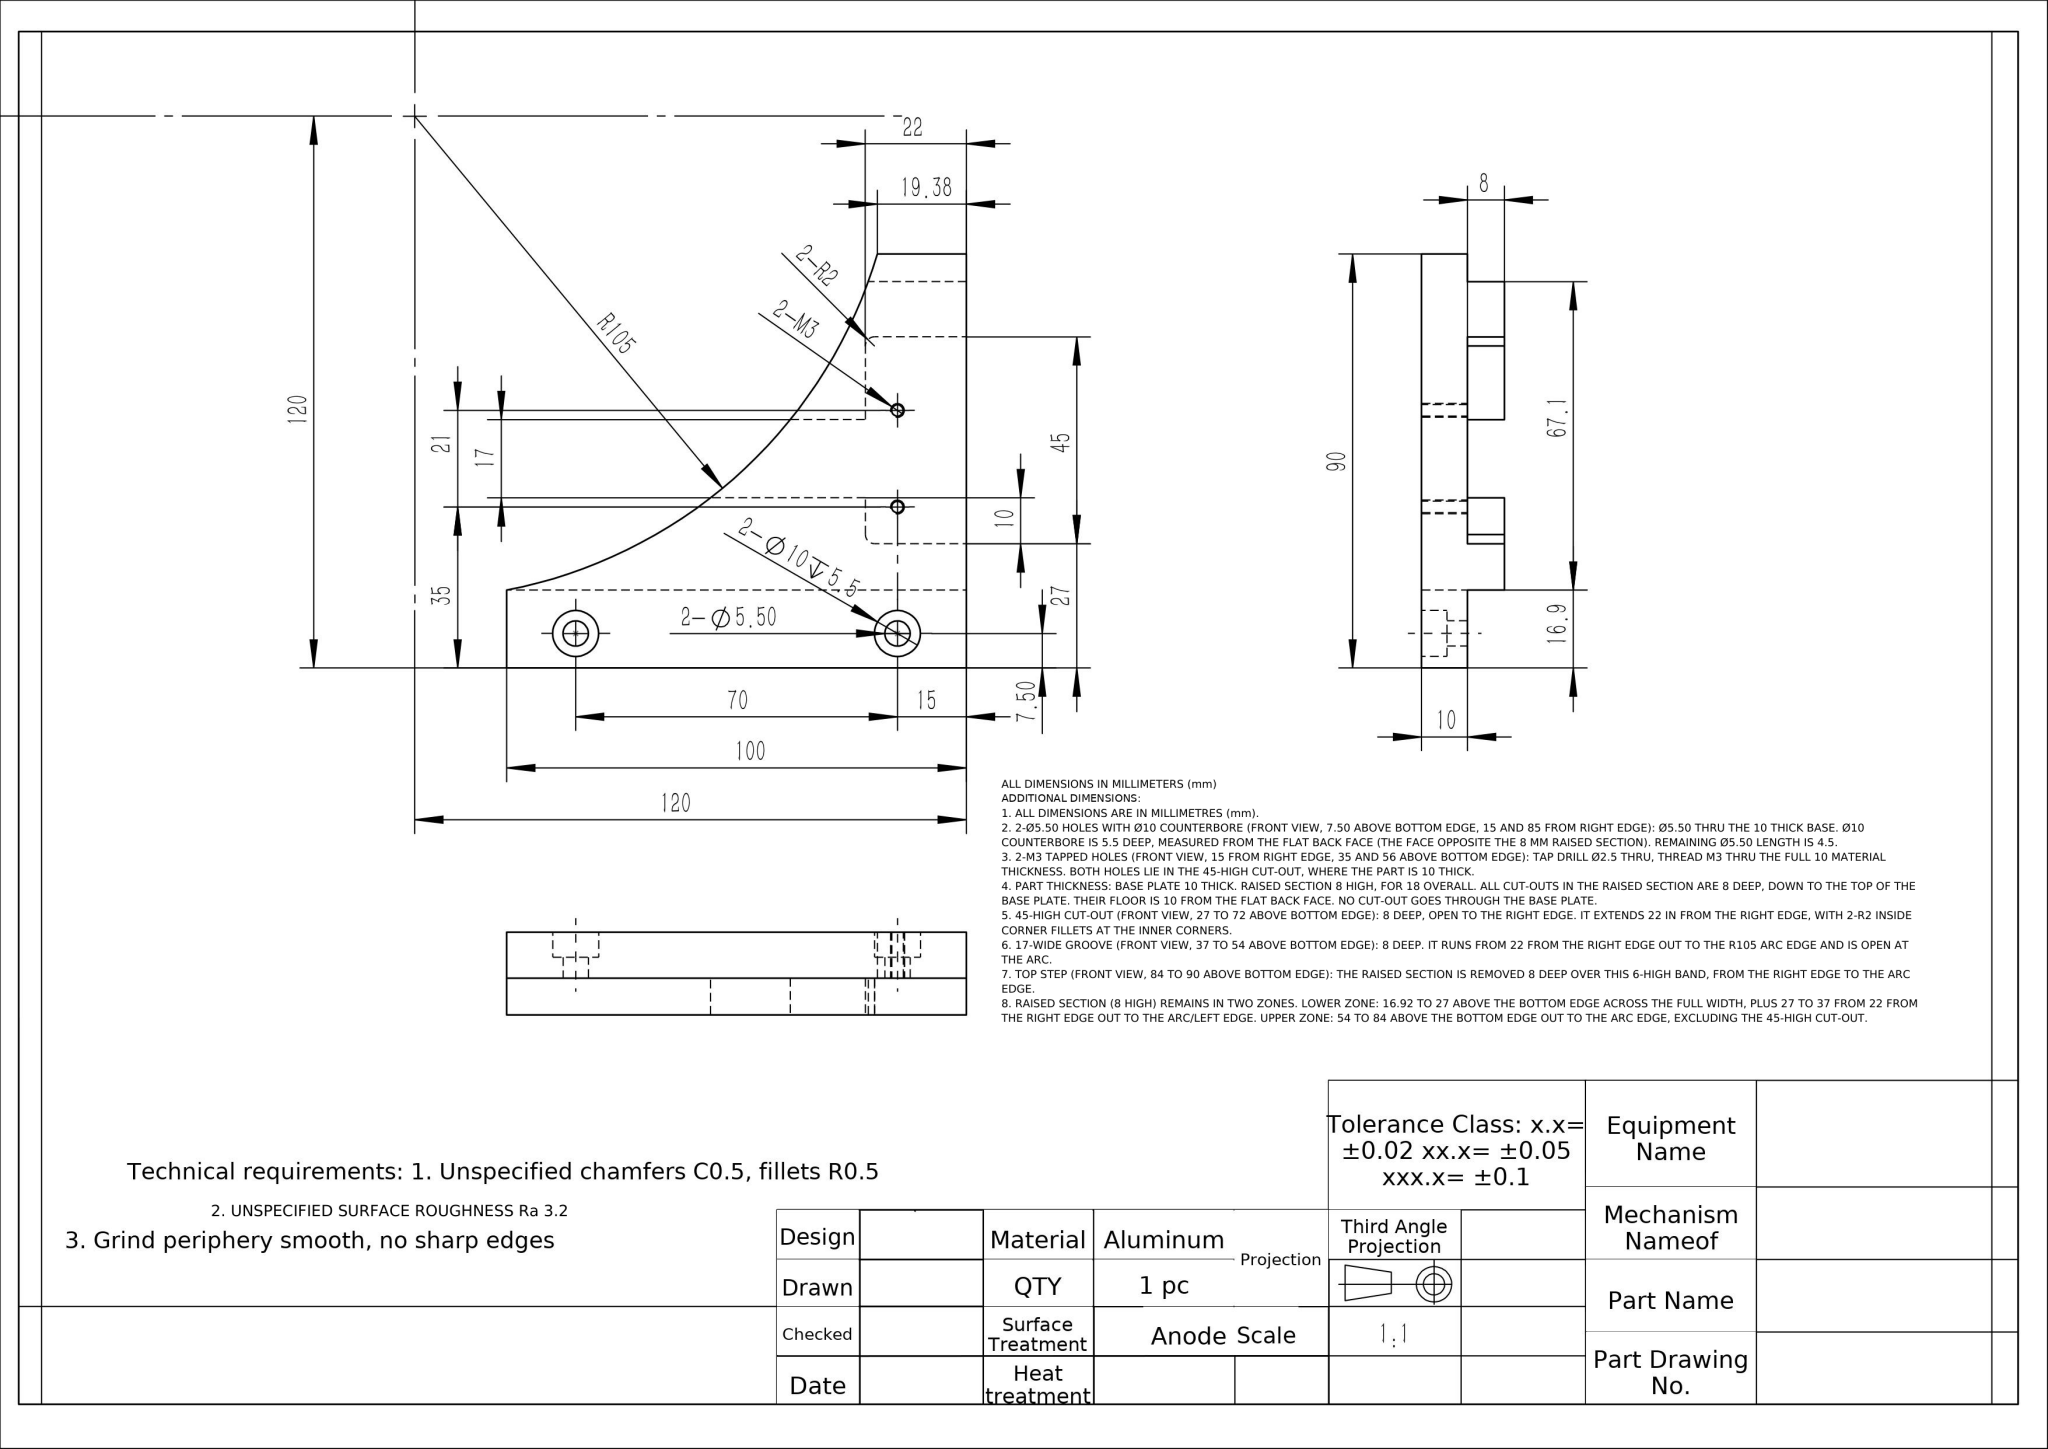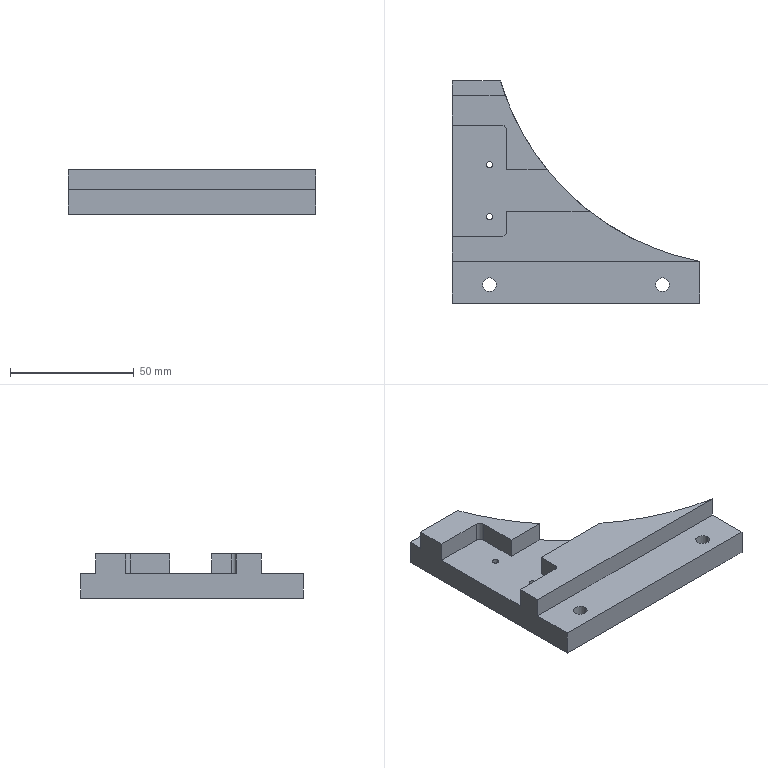Part | NX | mm | Stepped L-Shaped Three-Bore Bracket | 1 solid | 35 faces | box 100 x 90 x 18 mm | volume 61920 mm3 | plane 20 | cylinder 15 | commonest cylinder face diameters 10 x4 5.5 x4 2.5 x4 4 x2 210 x1